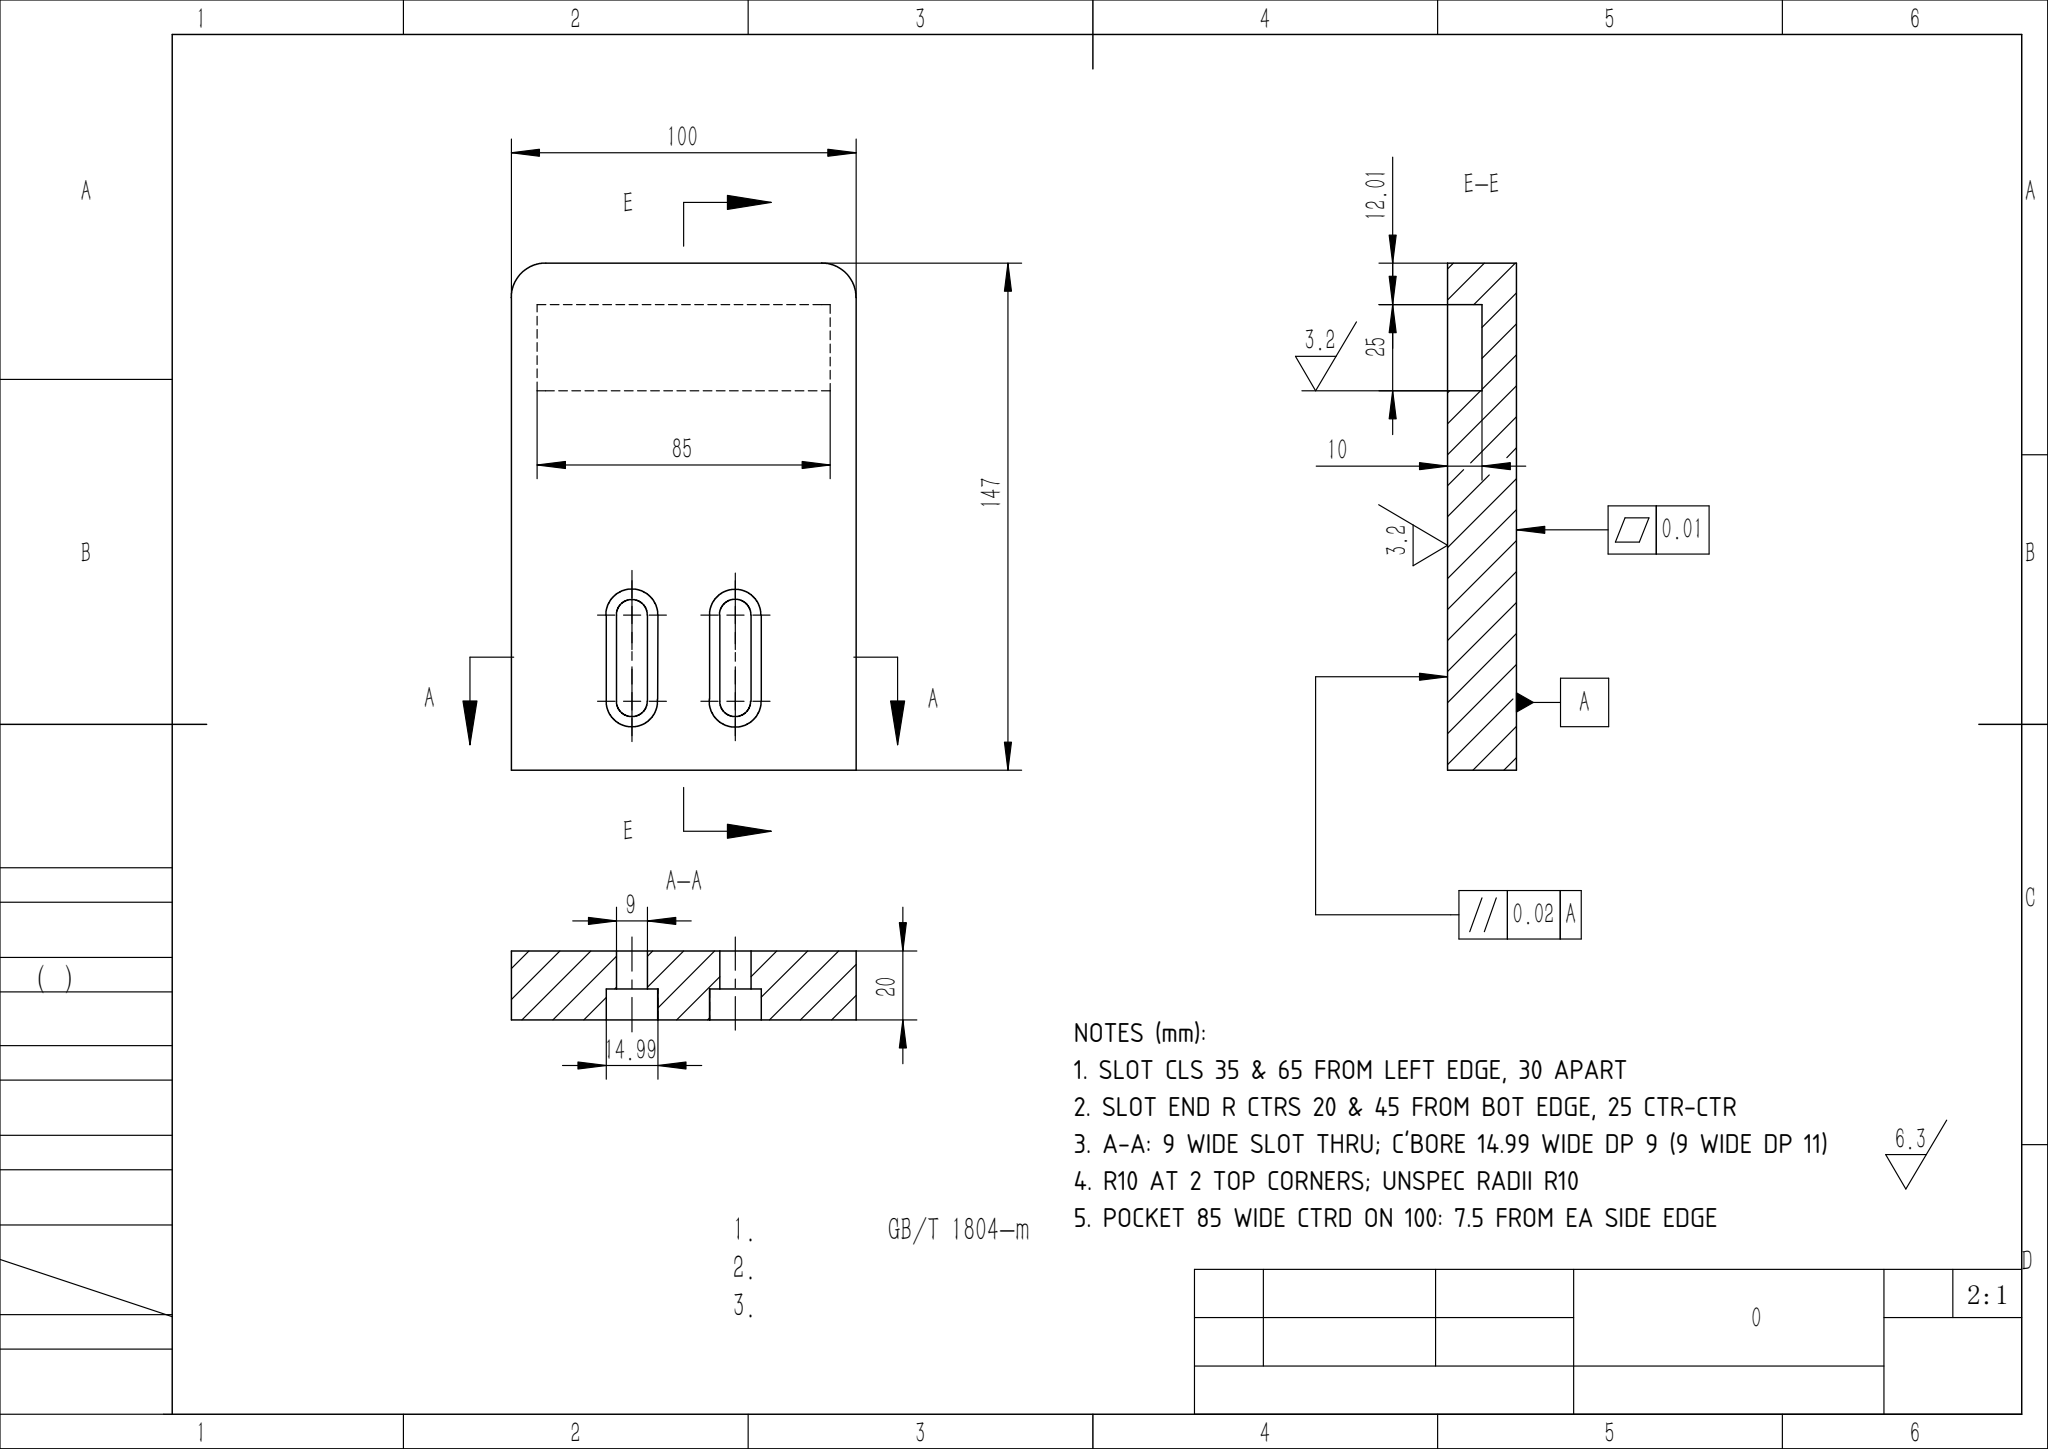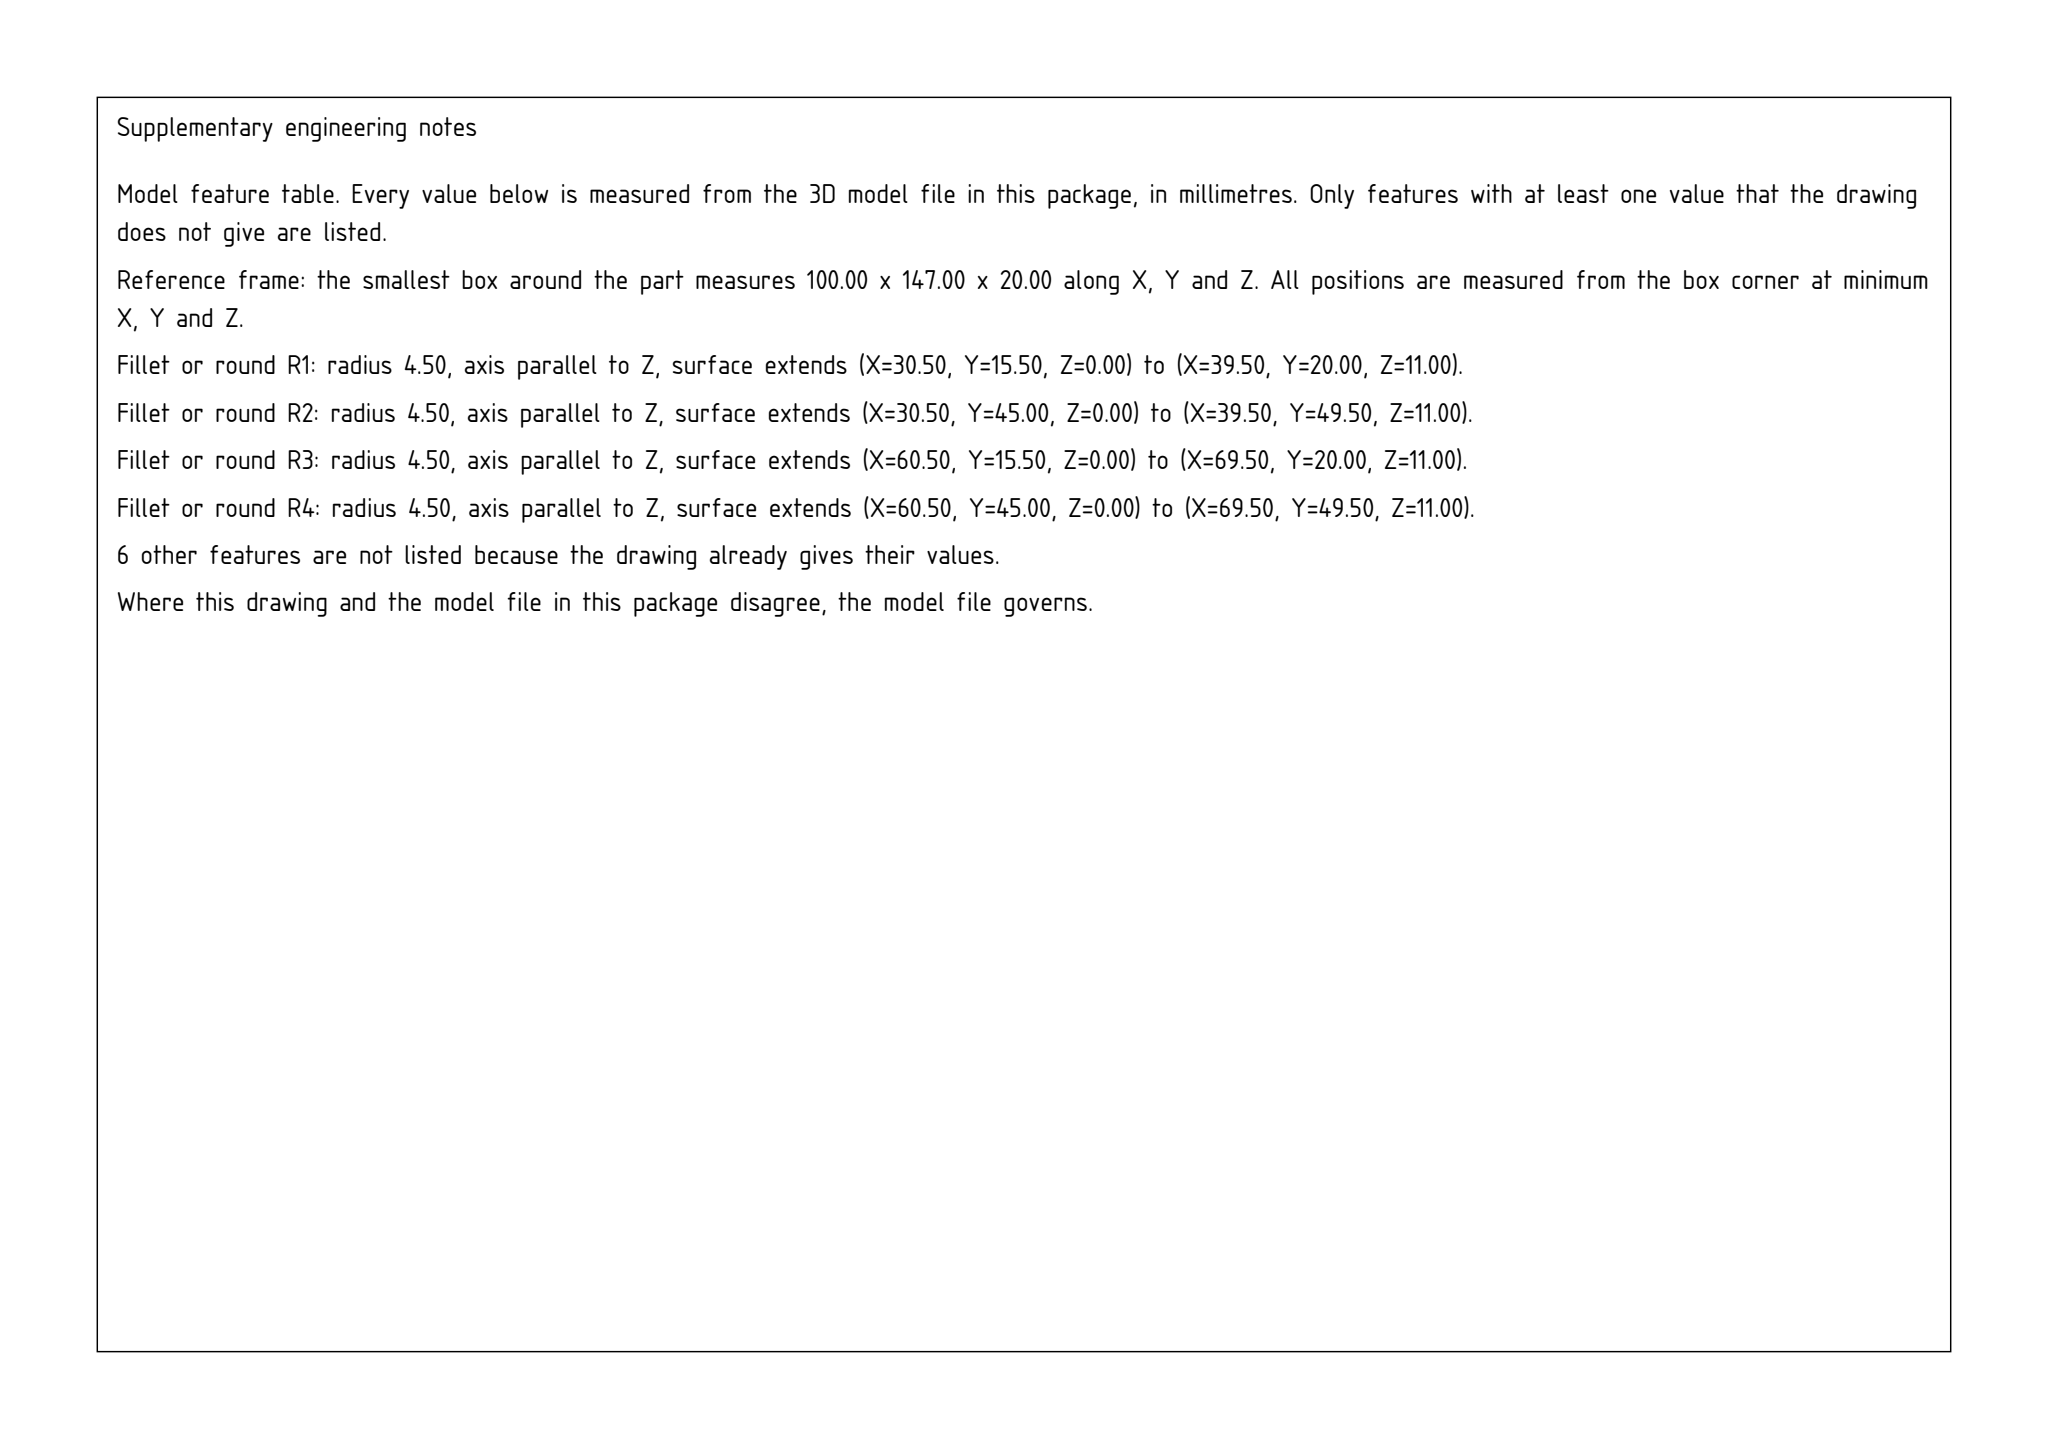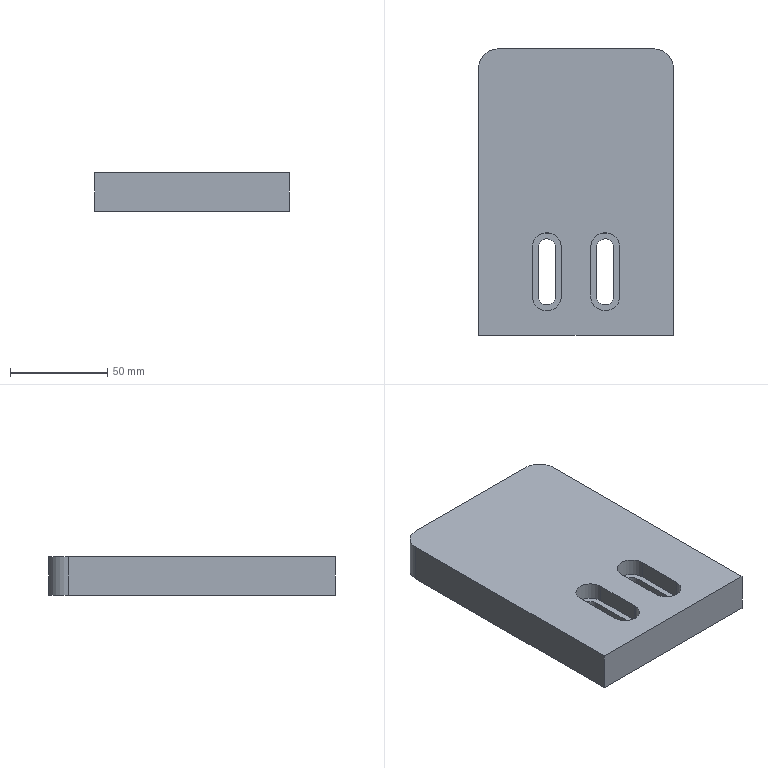Part | SolidWorks | mm | 1 solid | 32 faces | box 100 x 147 x 20 mm | volume 255617 mm3 | plane 21 | cylinder 11 | commonest cylinder face diameters 15 x5 9 x4 20 x2
Drawing notes:
SLOT CLS 35 & 65 FROM LEFT EDGE, 30 APART | from the solid: Ø15/Ø9 slot features at x=35 and x=65 of 100 wide bbox
SLOT END R CTRS 20 & 45 FROM BOT EDGE, 25 CTR-CTR | from the solid: slot cyl positions y=20 and y=45 of 147 tall bbox
A-A: 9 WIDE SLOT THRU; C'BORE 14.99 WIDE DP 9 (9 WIDE DP 11) | from the solid: Ø9 len 11 + Ø15 len 9 = 20 thk; z planes 0/11/20
R10 AT 2 TOP CORNERS; UNSPEC RADII R10 | from the solid: Ø20 z-cyls at (10,137) & (90,137) = R10 corners
POCKET 85 WIDE CTRD ON 100: 7.5 FROM EA SIDE EDGE | from the solid: x-planes at 7.5 and 92.5 bound 85-wide pocket in 100 bbox; 7.5 each side
build123d program:
from build123d import *

# Parameters (mm, degrees)
SKETCH1_W           = 100
SKETCH1_H           = 147
BOSS_EXTRUDE1_DEPTH = 20
CUT_EXTRUDE1_DEPTH  = 47
CUT_EXTRUDE2_DEPTH  = 9
FILLET1_R           = 10
SKETCH4_W           = 85
SKETCH4_H           = 25
CUT_EXTRUDE3_DEPTH  = 10


with BuildPart() as part:
    # Sketch1 → Boss-Extrude1 (new body)
    with BuildSketch(Plane.XY):
        Rectangle(SKETCH1_W, SKETCH1_H)
    extrude(amount=BOSS_EXTRUDE1_DEPTH)

    # Sketch2 → Cut-Extrude1 (cut)
    with BuildSketch(Plane.XY.offset(20)):
        with BuildLine():
            Line((-10.5, -28.5), (-10.5, -53.5))
            ThreePointArc((-10.5, -53.5), (-15, -58), (-19.5, -53.5))
            Line((-19.5, -53.5), (-19.5, -28.5))
            ThreePointArc((-19.5, -28.5), (-15, -24), (-10.5, -28.5))
        make_face()
    cut_extrude1 = extrude(amount=-CUT_EXTRUDE1_DEPTH, mode=Mode.SUBTRACT)

    # Mirror1: Cut-Extrude1 across plane
    add(cut_extrude1.mirror(Plane(origin=(0, 0, 0), x_dir=(0, 0, 1), z_dir=(1, 0, 0))), mode=Mode.SUBTRACT)

    # Sketch3 → Cut-Extrude2 (cut)
    with BuildSketch(Plane.XY.offset(20)):
        with BuildLine():
            Line((-7.5, -28.5), (-7.526, -52.873))
            ThreePointArc((-7.526, -52.873), (-14.686, -60.993), (-22.5, -53.5))
            Line((-22.5, -53.5), (-22.5, -28.5))
            ThreePointArc((-22.5, -28.5), (-15, -21), (-7.5, -28.5))
        make_face()
    cut_extrude2 = extrude(amount=-CUT_EXTRUDE2_DEPTH, mode=Mode.SUBTRACT)

    # Mirror2: Cut-Extrude2 across plane
    add(cut_extrude2.mirror(Plane(origin=(0, 0, 0), x_dir=(0, 0, 1), z_dir=(1, 0, 0))), mode=Mode.SUBTRACT)

    # Fillet1
    fillet1_edges = [part.edges().sort_by_distance(p)[0] for p in [
        (-50, 73.5, 10),
        (50, 73.5, 10),
    ]]
    fillet(fillet1_edges, radius=FILLET1_R)

    # Sketch4 → Cut-Extrude3 (cut)
    with BuildSketch(Plane(origin=(0, 0, 0), x_dir=(-1, 0, 0), z_dir=(0, 0, -1))):
        with Locations((0, 48.994)):
            Rectangle(SKETCH4_W, SKETCH4_H)
    extrude(amount=-CUT_EXTRUDE3_DEPTH, mode=Mode.SUBTRACT)


solid = part.part